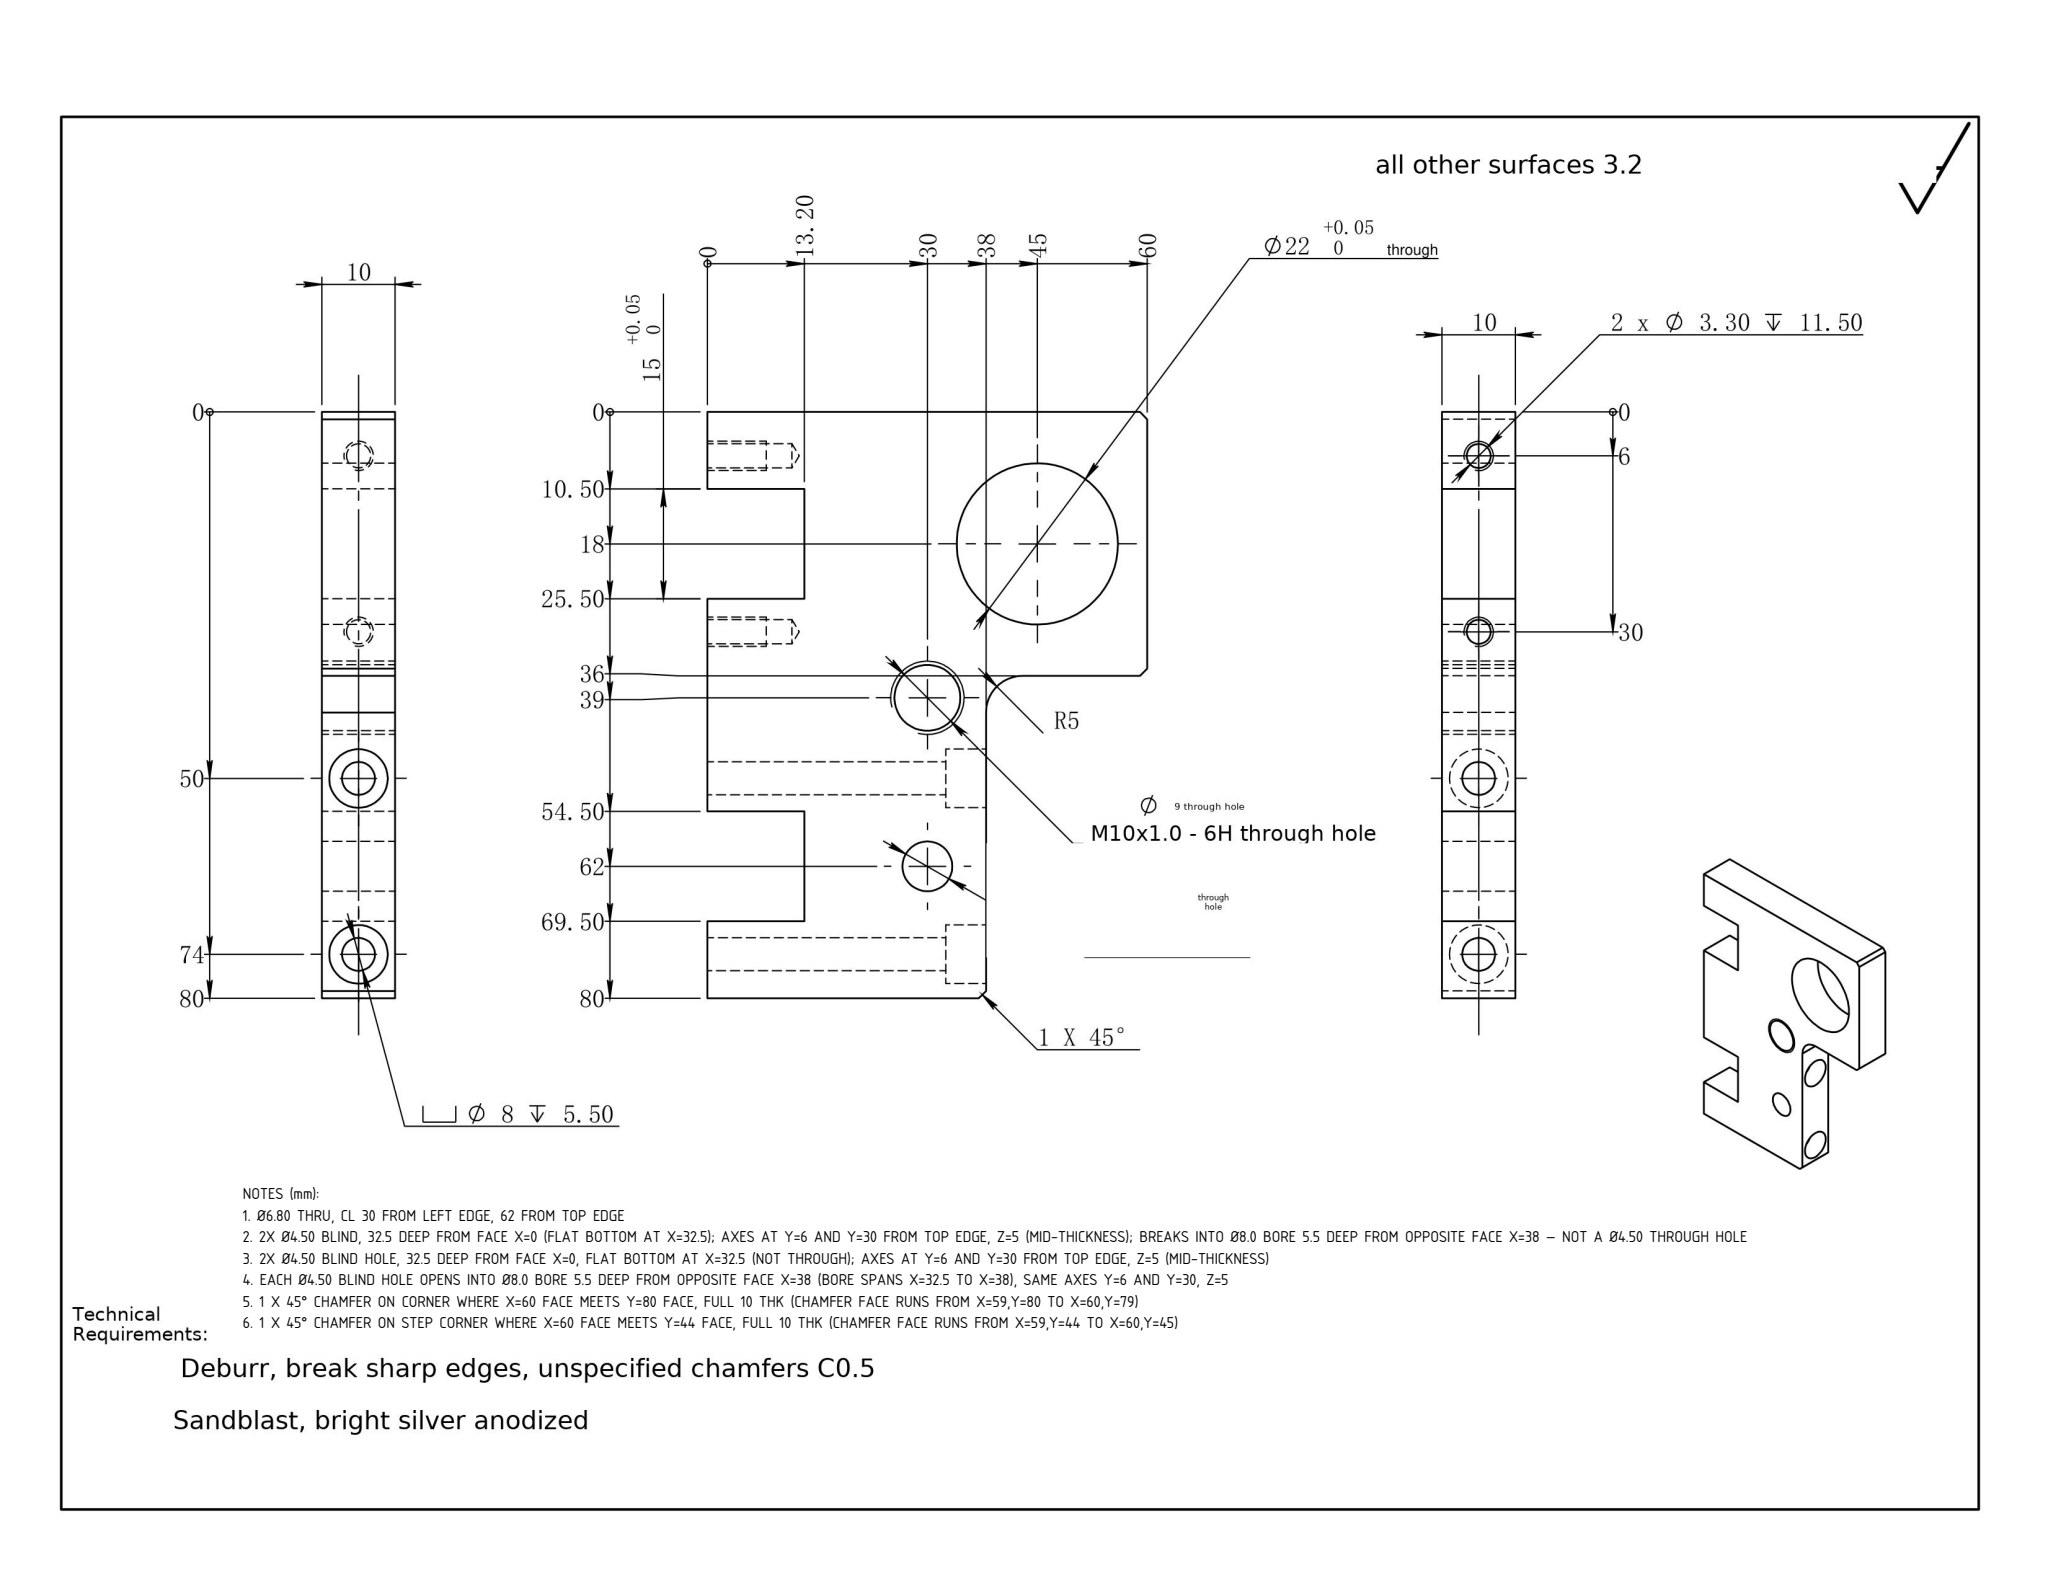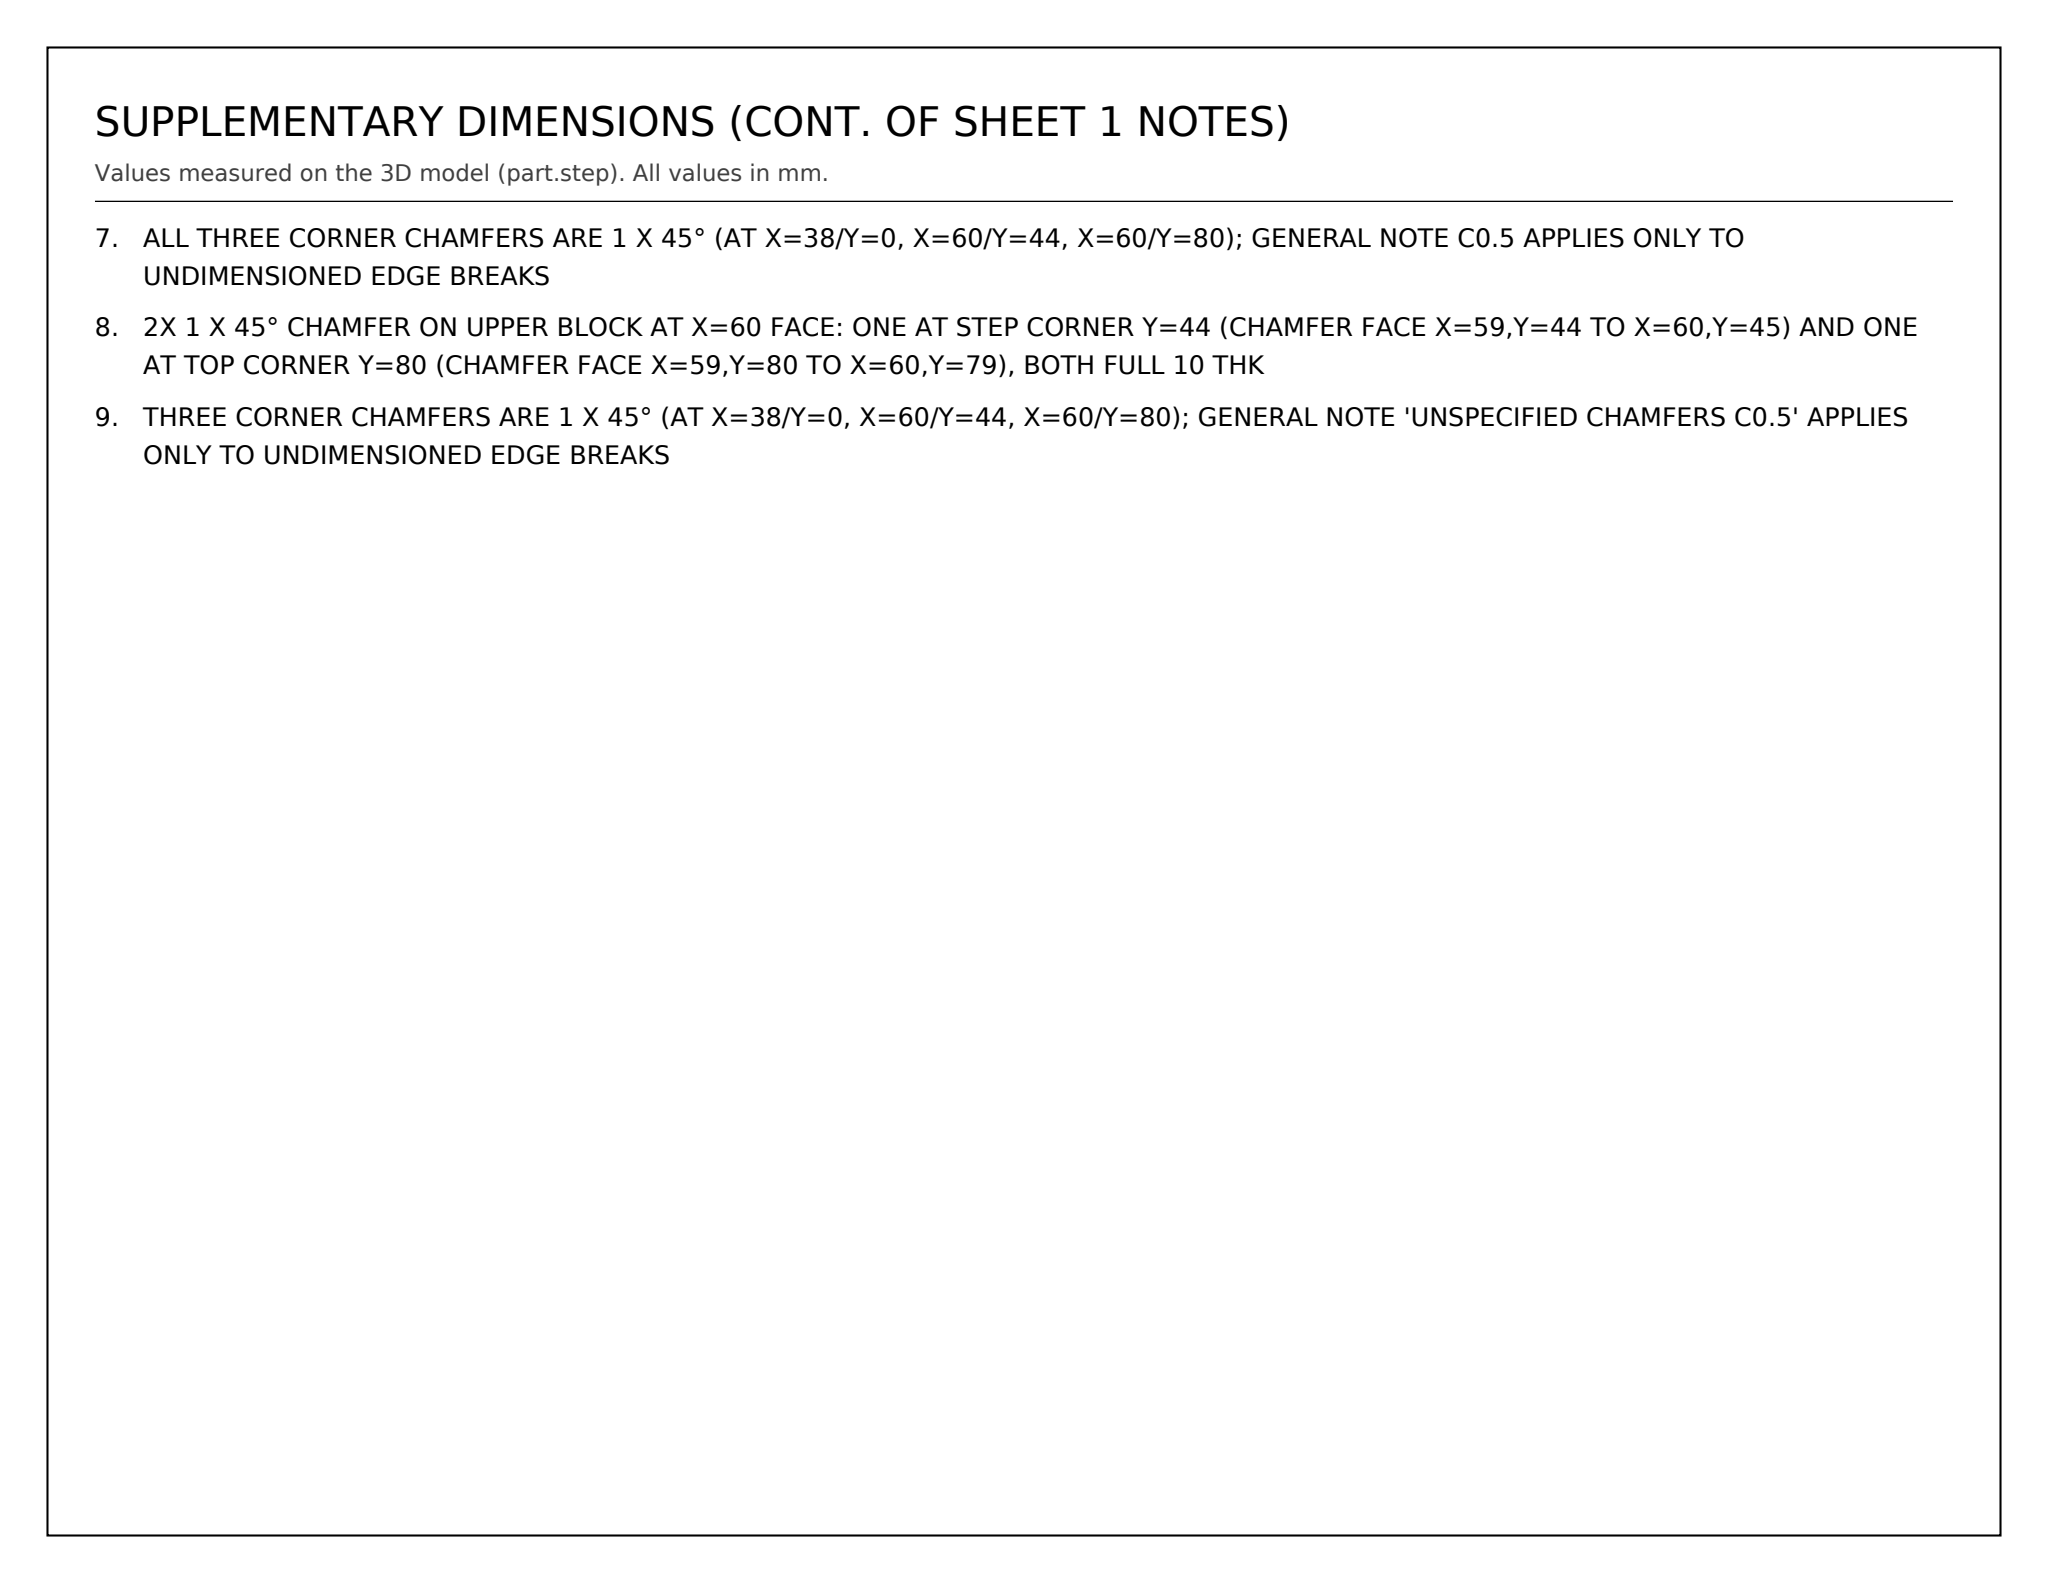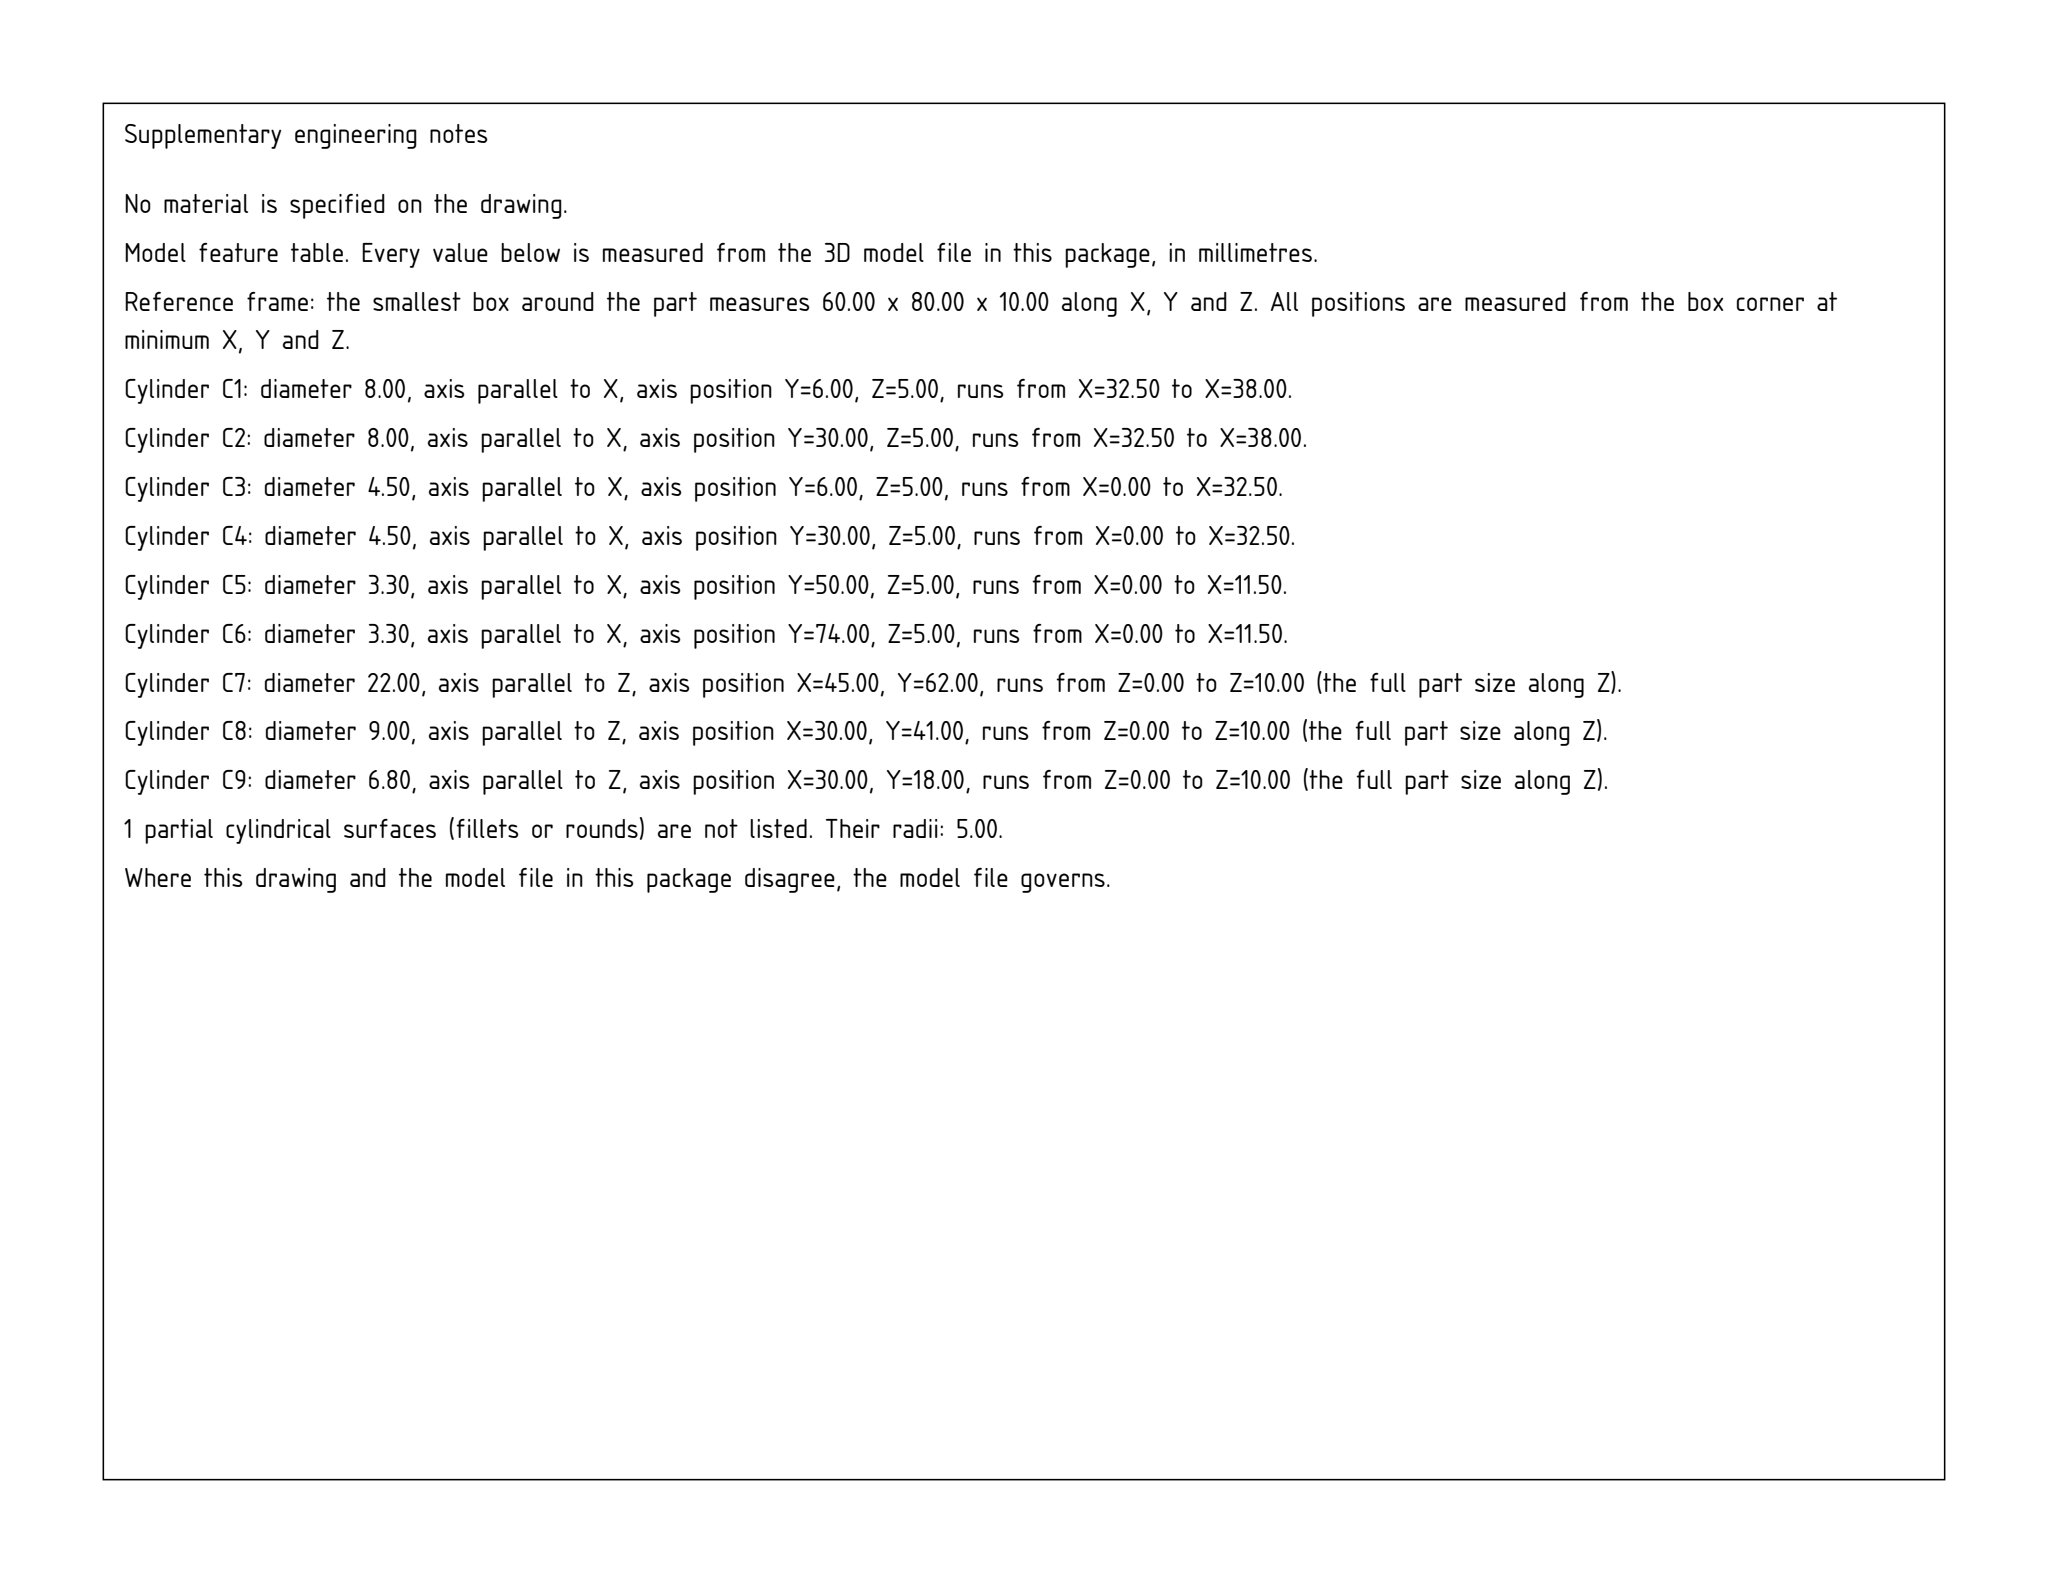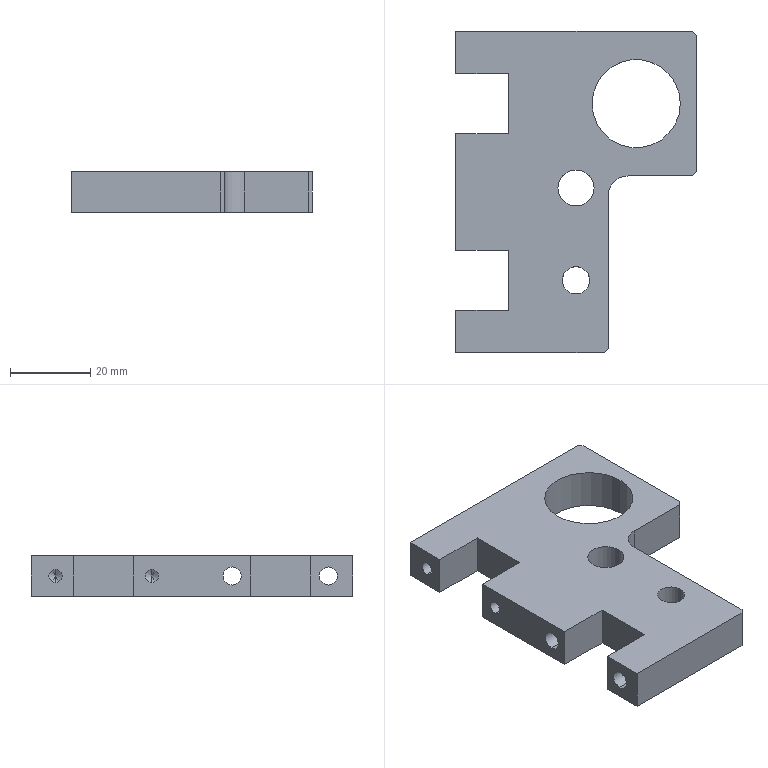Part | SolidWorks | mm | 1 solid | 44 faces | box 60 x 80 x 10 mm | volume 27809 mm3 | plane 21 | cylinder 19 | cone 4 | commonest cylinder face diameters 3.3 x4 8 x4 4.5 x4 6.8 x2 9 x2 22 x2 10 x1
Drawing notes:
Ø6.80 THRU, CL 30 FROM LEFT EDGE, 62 FROM TOP EDGE | from the solid: cyl dia 6.8 axis z at (x=30.0, y=18.0), len 10.0 = full thk; y=18 -> 62 from top datum
2X Ø4.50 BLIND, 32.5 DEEP FROM FACE X=0 (FLAT BOTTOM AT X=32.5); AXES AT Y=6 AND Y=30 FROM TOP EDGE, Z=5 (MID-THICKNESS); BREAKS INTO Ø8.0 BORE 5.5 DEEP FROM OPPOSITE FACE X=38 — NOT A Ø4.50 THROUGH HOLE | from the solid: cylinders: hole/bore 4.5 dia, axis x at (y=30, z=5) and (y=6, z=5), from 0.0 to 32.5; hole/bore 8.0 dia, axis x, same positions, from 32.5 to 38.0; axis_planes x=32.5 extents y[2,10] and y[26,34], z[1,9] (annular flat bottom)
2X Ø4.50 BLIND HOLE, 32.5 DEEP FROM FACE X=0, FLAT BOTTOM AT X=32.5 (NOT THROUGH); AXES AT Y=6 AND Y=30 FROM TOP EDGE, Z=5 (MID-THICKNESS) | from the solid: cylinders: hole/bore 4.5 dia, axis x, at (y=6,z=5) and (y=30,z=5), from 0.0 to 32.5; axis_planes x=32.5 extents y[2,10] and y[26,34], z[1,9] (flat bottoms)
EACH Ø4.50 BLIND HOLE OPENS INTO Ø8.0 BORE 5.5 DEEP FROM OPPOSITE FACE X=38 (BORE SPANS X=32.5 TO X=38), SAME AXES Y=6 AND Y=30, Z=5 | from the solid: cylinders: hole/bore 8.0 dia, axis x, at (y=6,z=5) and (y=30,z=5), from 32.5 to 38.0; axis_plane x=38.0 extent y[1,39], z[0,10]
1 X 45° CHAMFER ON CORNER WHERE X=60 FACE MEETS Y=80 FACE, FULL 10 THK (CHAMFER FACE RUNS FROM X=59,Y=80 TO X=60,Y=79) | from the solid: inclined_planes: angle_to_xyz_axes [45,45,90], bbox_from [59.0,79.0,0.0], size [1.0,1.0,10.0]
1 X 45° CHAMFER ON STEP CORNER WHERE X=60 FACE MEETS Y=44 FACE, FULL 10 THK (CHAMFER FACE RUNS FROM X=59,Y=44 TO X=60,Y=45) | from the solid: inclined_planes: angle_to_xyz_axes [45,45,90], bbox_from [59.0,44.0,0.0], size [1.0,1.0,10.0]
ALL THREE CORNER CHAMFERS ARE 1 X 45° (AT X=38/Y=0, X=60/Y=44, X=60/Y=80); GENERAL NOTE C0.5 APPLIES ONLY TO UNDIMENSIONED EDGE BREAKS | from the solid: inclined_planes: three 45° faces of size 1.0 x 1.0 x 10.0 at bbox_from [37,0,0], [59,44,0], [59,79,0]
2X 1 X 45° CHAMFER ON UPPER BLOCK AT X=60 FACE: ONE AT STEP CORNER Y=44 (CHAMFER FACE X=59,Y=44 TO X=60,Y=45) AND ONE AT TOP CORNER Y=80 (CHAMFER FACE X=59,Y=80 TO X=60,Y=79), BOTH FULL 10 THK | from the solid: inclined_planes: angle_to_xyz_axes [45,45,90], bbox_from [59.0,44.0,0.0] size [1,1,10]; and bbox_from [59.0,79.0,0.0] size [1,1,10]
THREE CORNER CHAMFERS ARE 1 X 45° (AT X=38/Y=0, X=60/Y=44, X=60/Y=80); GENERAL NOTE 'UNSPECIFIED CHAMFERS C0.5' APPLIES ONLY TO UNDIMENSIONED EDGE BREAKS | from the solid: inclined_planes: three 45° faces at bbox_from [37,0,0], [59,44,0], [59,79,0], each size [1,1,10]
build123d program:
from build123d import *

# Parameters (mm, degrees)
SKETCH1_W                                       = 80
SKETCH1_H                                       = 10
BOSS_EXTRUDE1_DEPTH                             = 60
SKETCH13_W                                      = 22
SKETCH13_H                                      = 44
CUT_EXTRUDE3_DEPTH                              = 73.801
M4_HEX_SOCKET_HEAD_CAP_SCREW_CBORE1_D           = 4.5
M4_HEX_SOCKET_HEAD_CAP_SCREW_CBORE1_CBORE_D     = 8
M4_HEX_SOCKET_HEAD_CAP_SCREW_CBORE1_CBORE_DEPTH = 5.5
SKETCH9_R                                       = 11
CUT_EXTRUDE2_DEPTH                              = 73.801
M10X1_0_TAPPED_HOLE1_D                          = 9
SKETCH6_W                                       = 26.4
SKETCH6_H                                       = 15
CUT_EXTRUDE1_DEPTH                              = 73.801
M8_TAPPED_HOLE1_D                               = 6.8
M4_TAPPED_HOLE1_D                               = 3.3
M4_TAPPED_HOLE1_DEPTH                           = 11.5
M4_TAPPED_HOLE1_TIP                             = 0.9914
CHAMFER1_SIZE                                   = 1
FILLET1_R                                       = 5


with BuildPart() as part:
    # Sketch1 → Boss-Extrude1 (new body)
    with BuildSketch(Plane(origin=(0, 0, 0), x_dir=(0, -1, 0), z_dir=(1, 0, 0))):
        Rectangle(SKETCH1_W, SKETCH1_H)
    extrude(amount=BOSS_EXTRUDE1_DEPTH)

    # Sketch13 → Cut-Extrude3 (cut, through all)
    with BuildSketch(Plane.XY.offset(5)):
        with Locations((49, -18)):
            Rectangle(SKETCH13_W, SKETCH13_H)
    extrude(amount=-CUT_EXTRUDE3_DEPTH, mode=Mode.SUBTRACT)

    # M4 Hex Socket Head Cap Screw CBORE1 (through all)
    with Locations(Plane(origin=(38, 0, 0), x_dir=(0, -1, 0), z_dir=(1, 0, 0))):
        with Locations((10, 0), (34, 0)):
            CounterBoreHole(M4_HEX_SOCKET_HEAD_CAP_SCREW_CBORE1_D / 2, M4_HEX_SOCKET_HEAD_CAP_SCREW_CBORE1_CBORE_D / 2, M4_HEX_SOCKET_HEAD_CAP_SCREW_CBORE1_CBORE_DEPTH)

    # Sketch9 → Cut-Extrude2 (cut, through all)
    with BuildSketch(Plane.XY.offset(5)):
        with Locations((45, 22)):
            Circle(SKETCH9_R)
    extrude(amount=-CUT_EXTRUDE2_DEPTH, mode=Mode.SUBTRACT)

    # M10x1.0 Tapped Hole1 (through all)
    with Locations(Plane.XY.offset(5)):
        with Locations((30, 1)):
            Hole(M10X1_0_TAPPED_HOLE1_D / 2)

    # Sketch6 → Cut-Extrude1 (cut, through all)
    with BuildSketch(Plane.XY.offset(5)):
        with Locations((0, 22)):
            Rectangle(SKETCH6_W, SKETCH6_H)
        with Locations((0, -22)):
            Rectangle(SKETCH6_W, SKETCH6_H)
    extrude(amount=-CUT_EXTRUDE1_DEPTH, mode=Mode.SUBTRACT)

    # M8 Tapped Hole1 (through all)
    with Locations(Plane.XY.offset(5)):
        with Locations((30, -22)):
            Hole(M8_TAPPED_HOLE1_D / 2)

    # M4 Tapped Hole1
    with Locations(Plane.ZY):
        with Locations((0, 10), (0, 34)):
            Hole(M4_TAPPED_HOLE1_D / 2, depth=M4_TAPPED_HOLE1_DEPTH)
            with Locations((0, 0, -(M4_TAPPED_HOLE1_DEPTH + M4_TAPPED_HOLE1_TIP / 2))):  # 118° drill point
                Cone(0, M4_TAPPED_HOLE1_D / 2, M4_TAPPED_HOLE1_TIP, mode=Mode.SUBTRACT)

    # Chamfer1
    chamfer1_edges = [part.edges().sort_by_distance(p)[0] for p in [
        (60, 40, 0),
        (60, 4, 0),
        (38, -40, 0),
    ]]
    chamfer(chamfer1_edges, length=CHAMFER1_SIZE)

    # Fillet1
    fillet1_edges = [part.edges().sort_by_distance(p)[0] for p in [
        (38, 4, 0),
    ]]
    fillet(fillet1_edges, radius=FILLET1_R)


solid = part.part